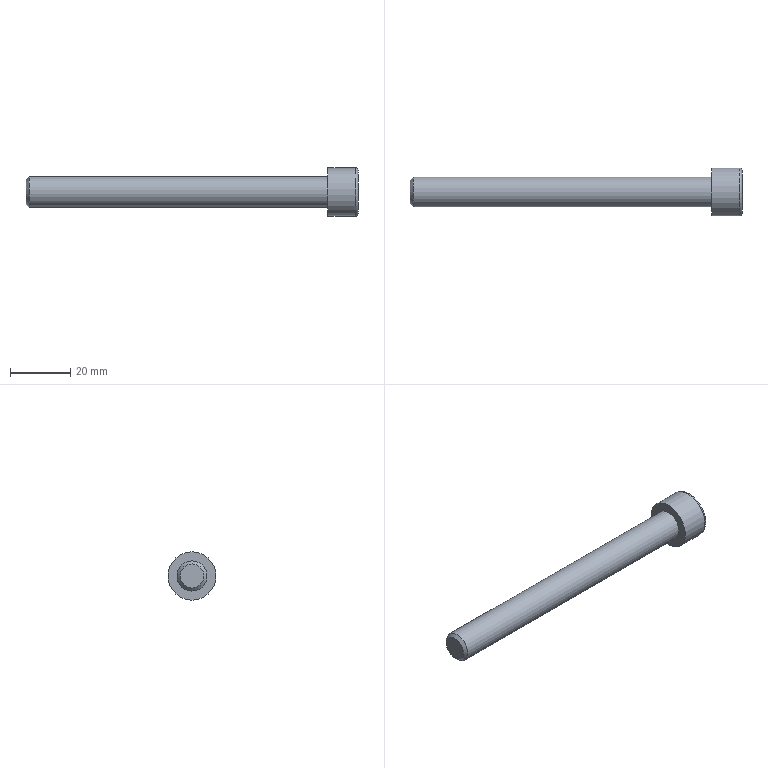Component | NX | GB_T70_1_M10X100_2 | 1 solid | 20 faces | volume 9435 mm3 | plane 15 | cylinder 2 | cone 2 | torus 1 | commonest cylinder face diameters 16 x1 10 x1